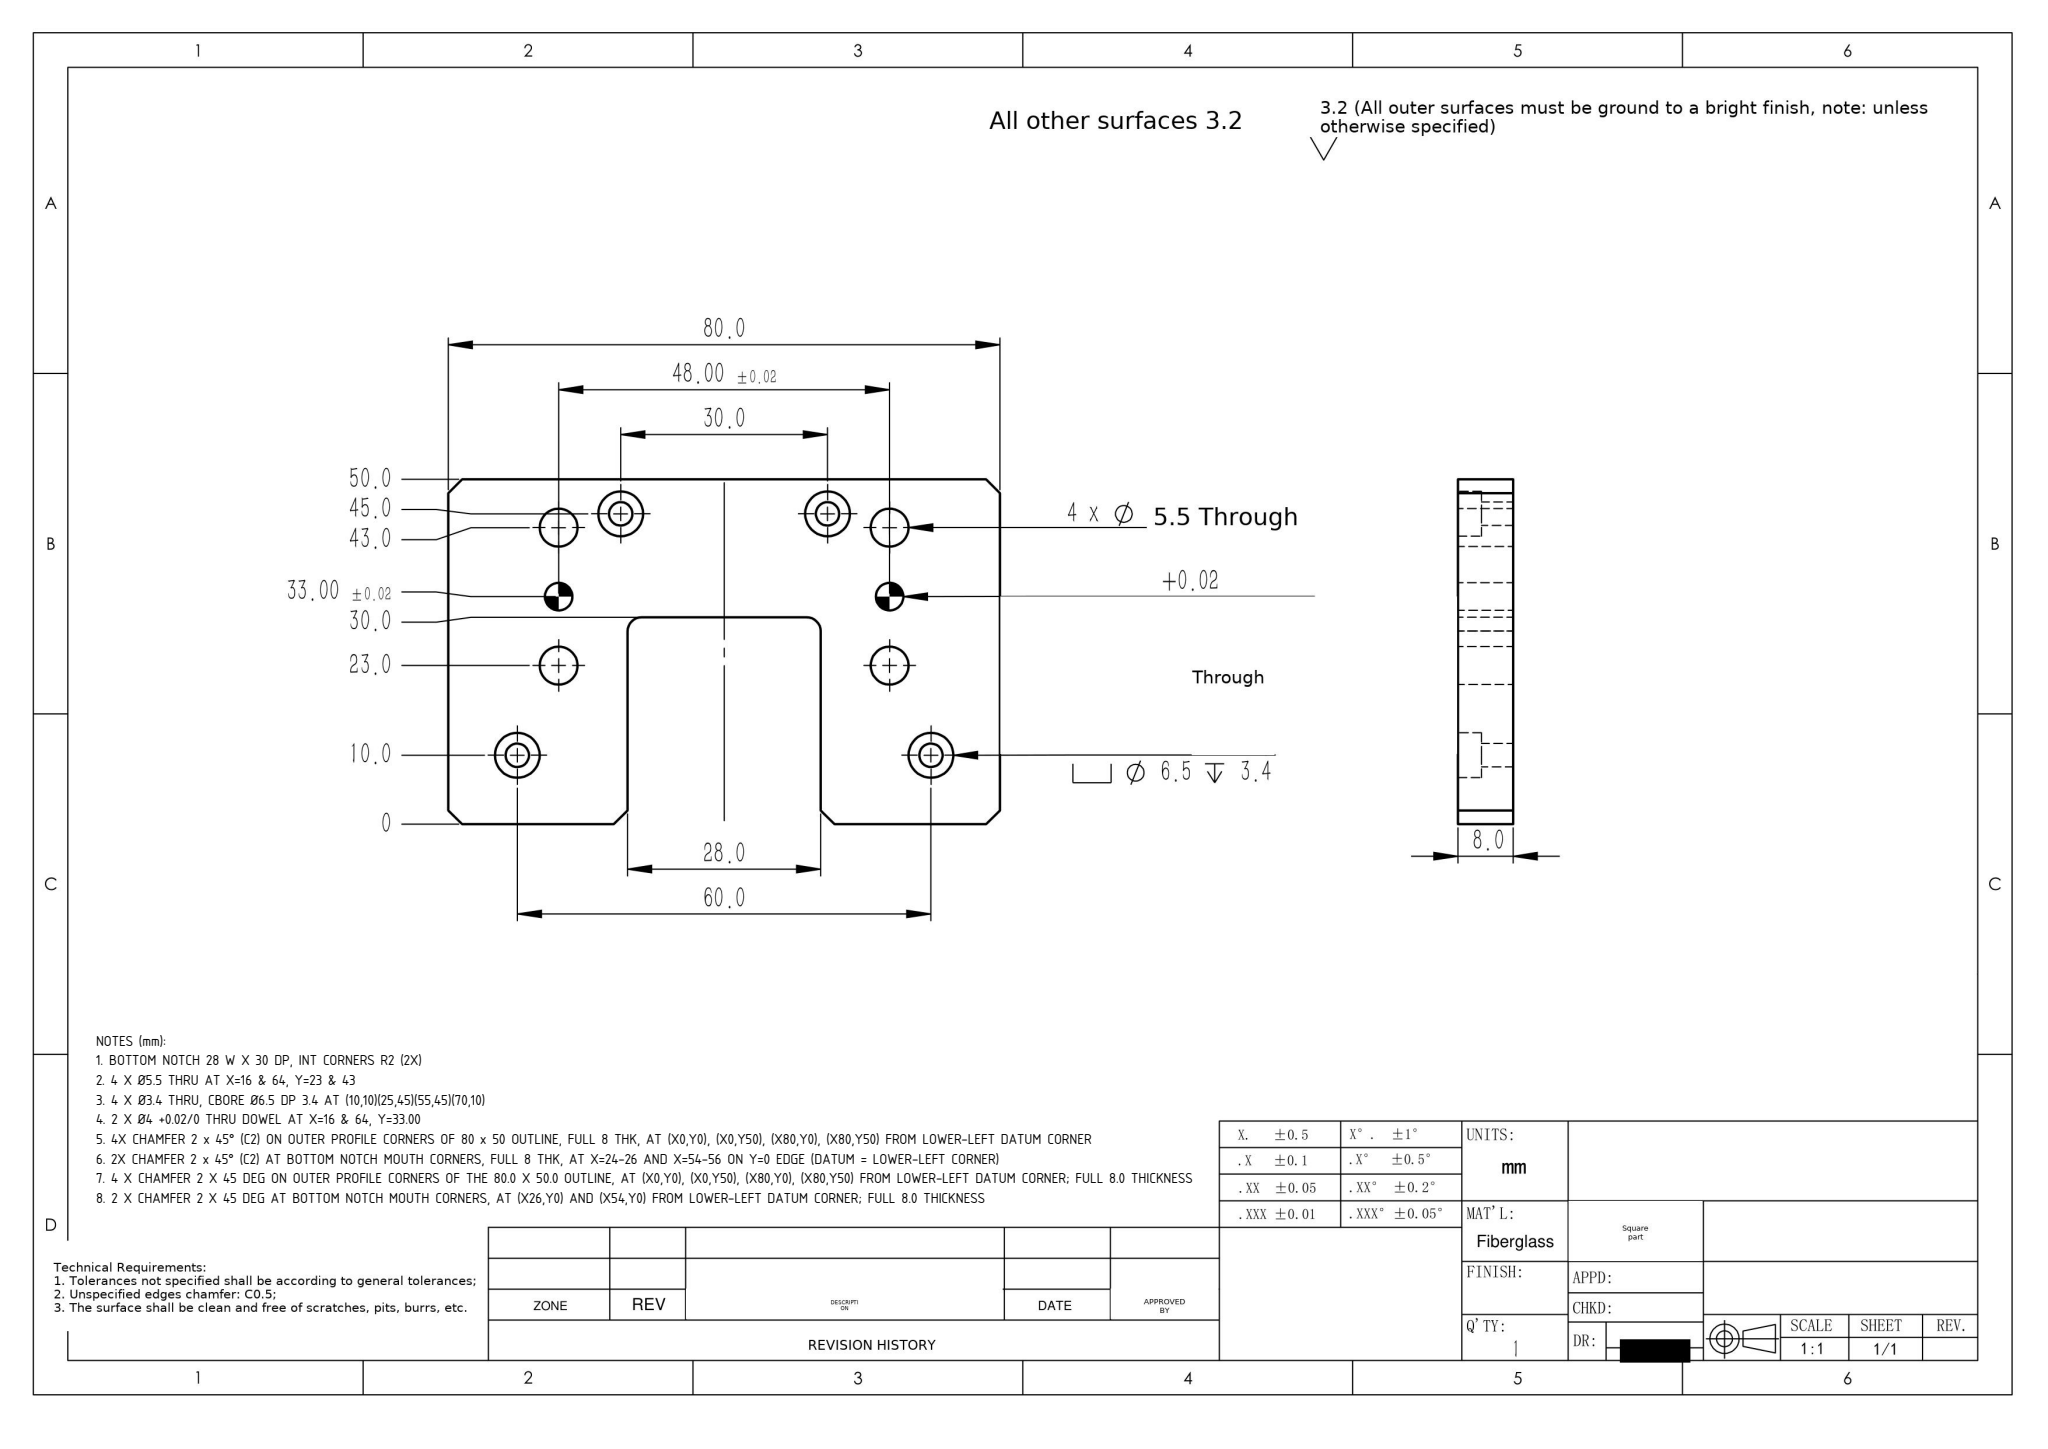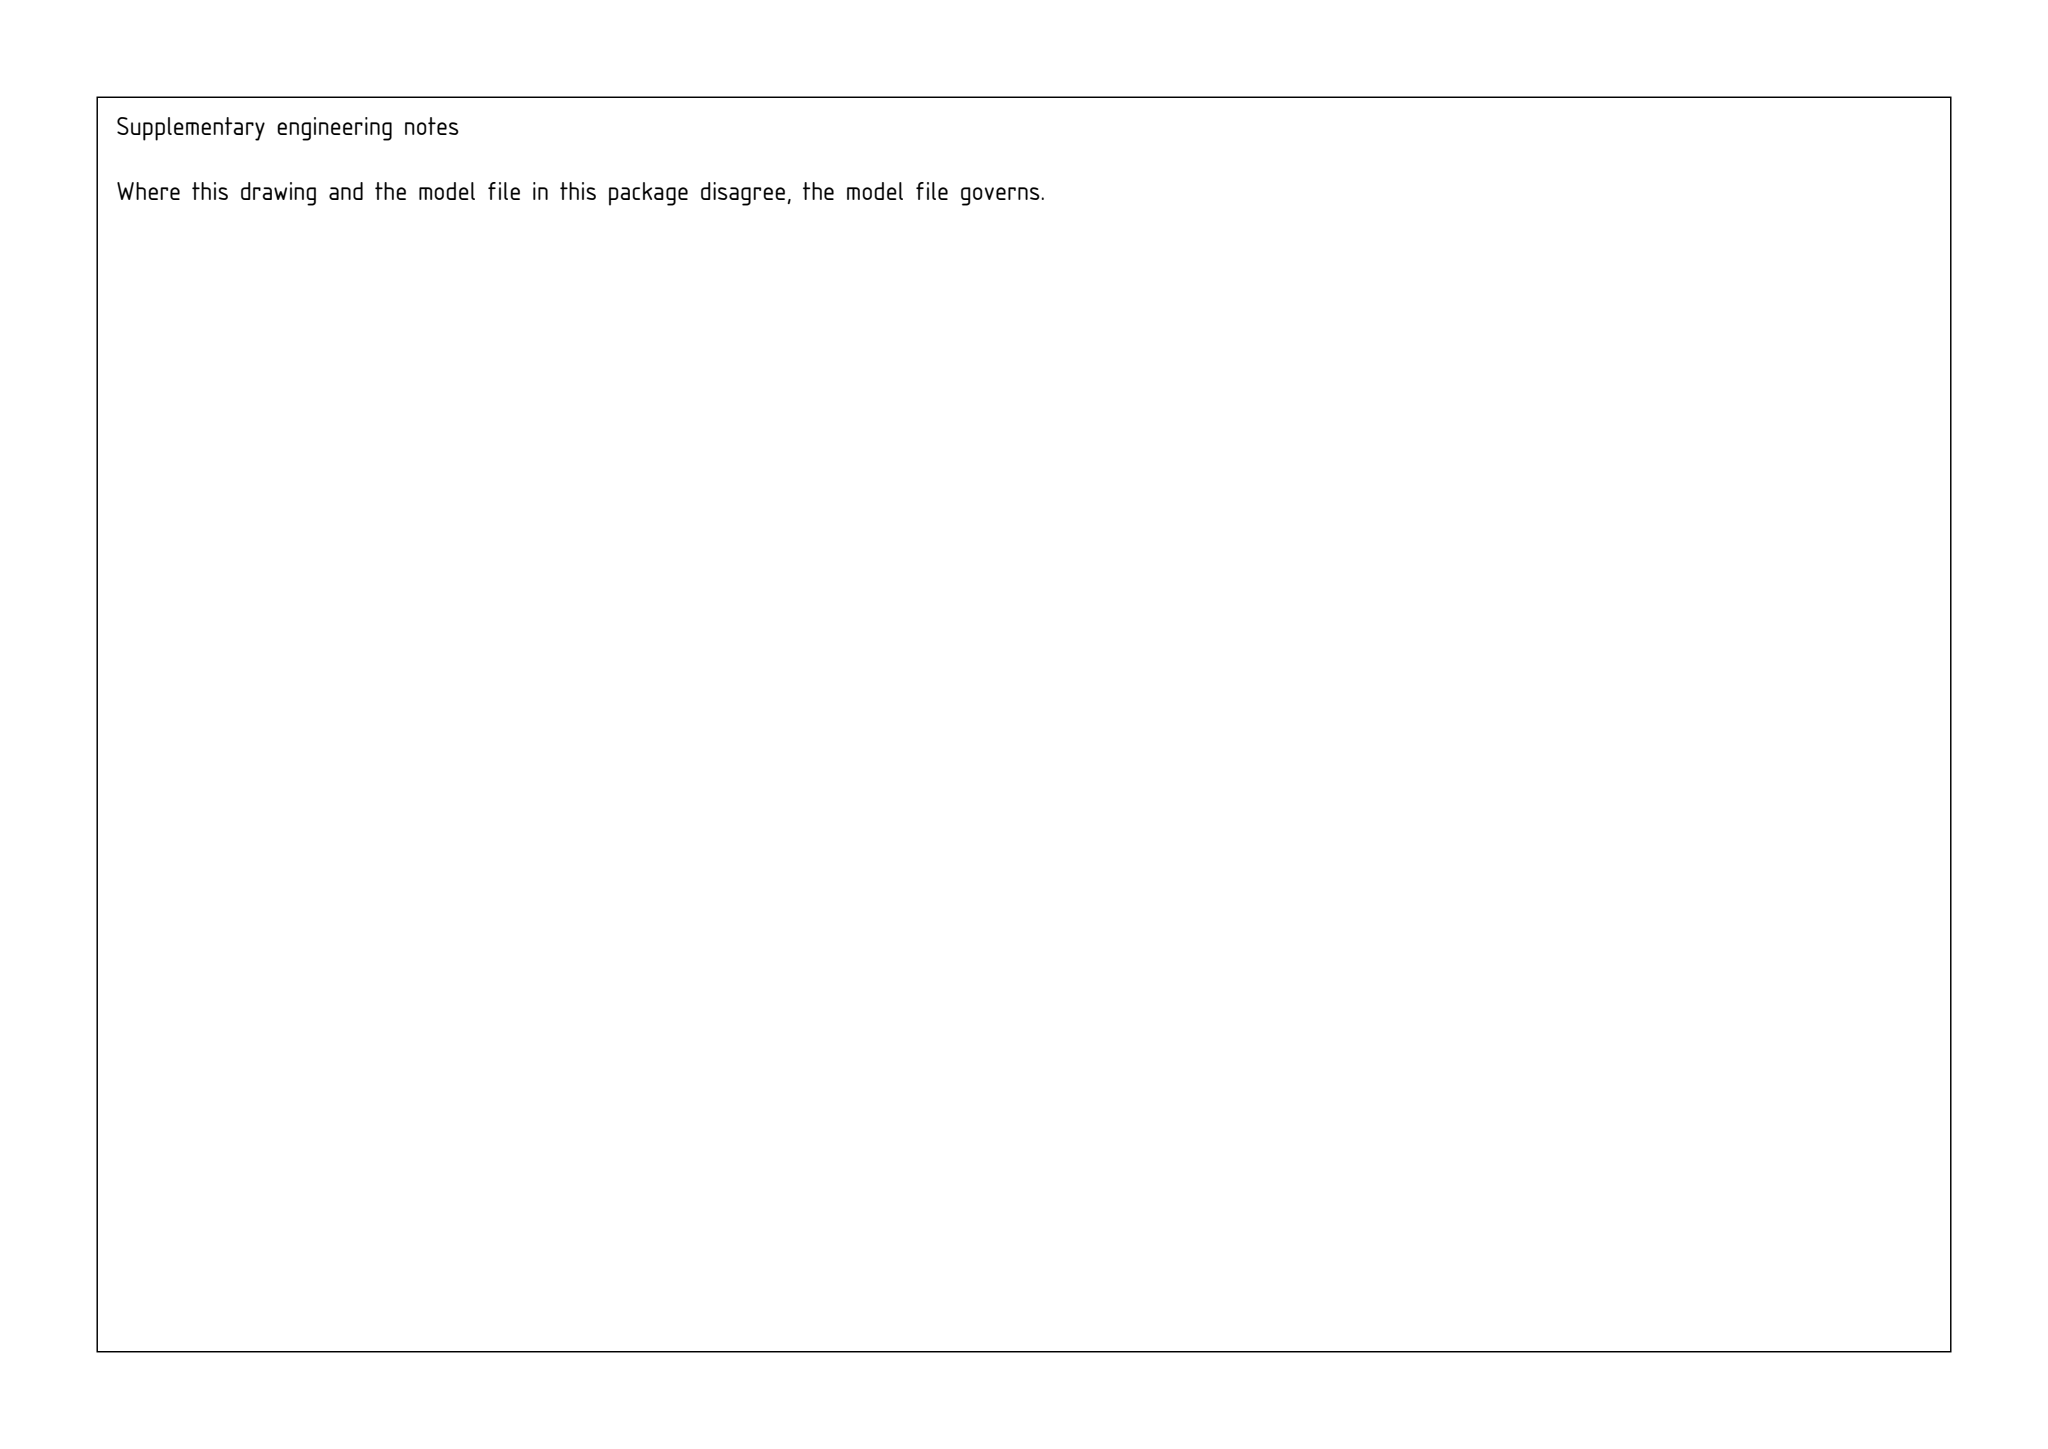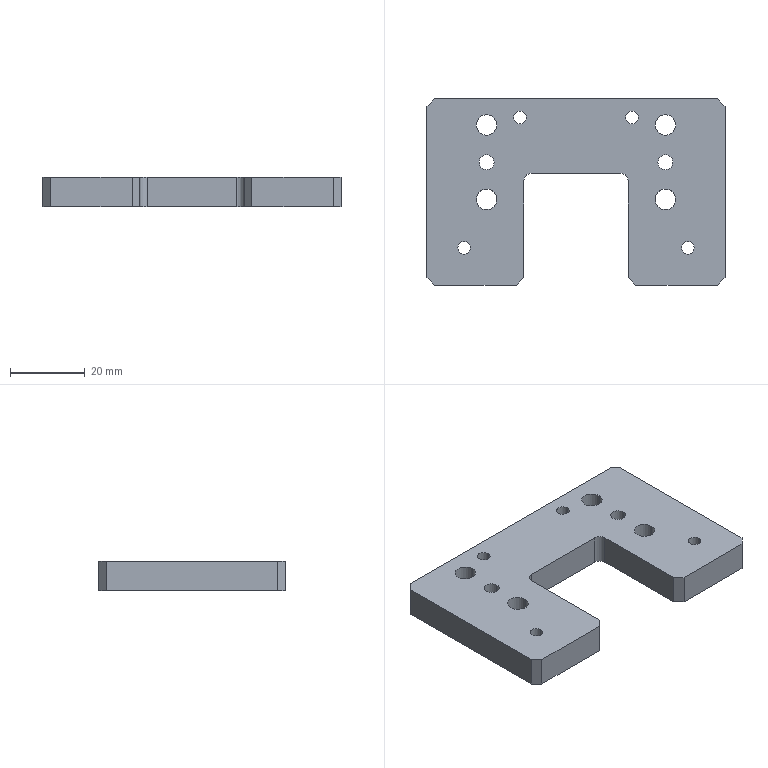Part | SolidWorks | mm | 1 solid | 50 faces | box 80 x 50 x 8 mm | volume 23618 mm3 | cylinder 30 | plane 20 | commonest cylinder face diameters 6.5 x8 3.4 x8 5.5 x8 4 x6
Drawing notes:
BOTTOM NOTCH 28 W X 30 DP, INT CORNERS R2 (2X) | from the solid: planes x=26 & x=54 (28 apart), y=0 to y=30; Ø4 z-cyl full 8 thru at (28,28) & (52,28) = R2 corners
4 X Ø5.5 THRU AT X=16 & 64, Y=23 & 43 | from the solid: dia 5.5 axis z at (16,23)(16,43)(64,23)(64,43), length 8.0 = full thk
4 X Ø3.4 THRU, CBORE Ø6.5 DP 3.4 AT (10,10)(25,45)(55,45)(70,10) | from the solid: dia 3.4 L4.6 at those pos with dia 6.5 L3.4 cbores; z=3.4 planes (4X)
2 X Ø4 +0.02/0 THRU DOWEL AT X=16 & 64, Y=33.00 | from the solid: dia 4.0 axis z at (16,33) & (64,33), length 8.0 = full thk
4X CHAMFER 2 x 45° (C2) ON OUTER PROFILE CORNERS OF 80 x 50 OUTLINE, FULL 8 THK, AT (X0,Y0), (X0,Y50), (X80,Y0), (X80,Y50) FROM LOWER-LEFT DATUM CORNER | from the solid: inclined_planes: four 45.0/45.0/90.0 faces, size 2.0 x 2.0 x 8.0, bbox_from [0,0,0], [0,48,0], [78,0,0], [78,48,0]
2X CHAMFER 2 x 45° (C2) AT BOTTOM NOTCH MOUTH CORNERS, FULL 8 THK, AT X=24-26 AND X=54-56 ON Y=0 EDGE (DATUM = LOWER-LEFT CORNER) | from the solid: inclined_planes: two 45.0/45.0/90.0 faces, size 2.0 x 2.0 x 8.0, bbox_from [24,0,0] and [54,0,0]; adjacent planes y=0 extent x[2,24] & x[56,78], x=26 and x=54 notch walls
4 X CHAMFER 2 X 45 DEG ON OUTER PROFILE CORNERS OF THE 80.0 X 50.0 OUTLINE, AT (X0,Y0), (X0,Y50), (X80,Y0), (X80,Y50) FROM LOWER-LEFT DATUM CORNER; FULL 8.0 THICKNESS | from the solid: inclined_planes 45/45/90, size [2,2,8] at bbox_from [0,0,0], [0,48,0], [78,0,0], [78,48,0] with bbox_xyz 80x50x8
2 X CHAMFER 2 X 45 DEG AT BOTTOM NOTCH MOUTH CORNERS, AT (X26,Y0) AND (X54,Y0) FROM LOWER-LEFT DATUM CORNER; FULL 8.0 THICKNESS | from the solid: inclined_planes 45/45/90, size [2,2,8] at bbox_from [24,0,0] and [54,0,0]; notch walls are planes x=26 and x=54 (y 2 to 28)
build123d program:
from build123d import *

# Parameters (mm, degrees)
SKETCH1_W                                       = 80
SKETCH1_H                                       = 50
BOSS_EXTRUDE1_DEPTH                             = 8
M5_CLEARANCE_HOLE1_D                            = 5.5
SIZE_MM_DOWEL_PIN_HOLE1_D                       = 4
SKETCH6_W                                       = 28
SKETCH6_H                                       = 30
CUT_EXTRUDE1_DEPTH                              = 65.529
M3_HEX_SOCKET_HEAD_CAP_SCREW_CBORE1_D           = 3.4
M3_HEX_SOCKET_HEAD_CAP_SCREW_CBORE1_CBORE_D     = 6.5
M3_HEX_SOCKET_HEAD_CAP_SCREW_CBORE1_CBORE_DEPTH = 3.4
CHAMFER1_SIZE                                   = 2
FILLET1_R                                       = 2


with BuildPart() as part:
    # Sketch1 → Boss-Extrude1 (new body)
    with BuildSketch(Plane.XY):
        with Locations((0, -25)):
            Rectangle(SKETCH1_W, SKETCH1_H)
    extrude(amount=BOSS_EXTRUDE1_DEPTH)

    # M5 Clearance Hole1 (through all)
    with Locations(Plane.XY.offset(8)):
        with Locations((-24, -7), (24, -7), (24, -27), (-24, -27)):
            Hole(M5_CLEARANCE_HOLE1_D / 2)

    # Size mm Dowel Pin Hole1 (through all)
    with Locations(Plane.XY.offset(8)):
        with Locations((-24, -17), (24, -17)):
            Hole(SIZE_MM_DOWEL_PIN_HOLE1_D / 2)

    # Sketch6 → Cut-Extrude1 (cut, through all)
    with BuildSketch(Plane.XY.offset(8)):
        with Locations((0, -35)):
            Rectangle(SKETCH6_W, SKETCH6_H)
    extrude(amount=-CUT_EXTRUDE1_DEPTH, mode=Mode.SUBTRACT)

    # M3 Hex Socket Head Cap Screw CBORE1 (through all)
    with Locations(Plane(origin=(0, 0, 0), x_dir=(-1, 0, 0), z_dir=(0, 0, -1))):
        with Locations((-30, -40), (30, -40), (-15, -5), (15, -5)):
            CounterBoreHole(M3_HEX_SOCKET_HEAD_CAP_SCREW_CBORE1_D / 2, M3_HEX_SOCKET_HEAD_CAP_SCREW_CBORE1_CBORE_D / 2, M3_HEX_SOCKET_HEAD_CAP_SCREW_CBORE1_CBORE_DEPTH)

    # Chamfer1
    chamfer1_edges = [part.edges().sort_by_distance(p)[0] for p in [
        (-14, -50, 4),
        (14, -50, 4),
        (-40, 0, 4),
        (40, 0, 4),
        (40, -50, 4),
        (-40, -50, 4),
    ]]
    chamfer(chamfer1_edges, length=CHAMFER1_SIZE)

    # Fillet1
    fillet1_edges = [part.edges().sort_by_distance(p)[0] for p in [
        (-14, -20, 4),
        (14, -20, 4),
    ]]
    fillet(fillet1_edges, radius=FILLET1_R)


solid = part.part